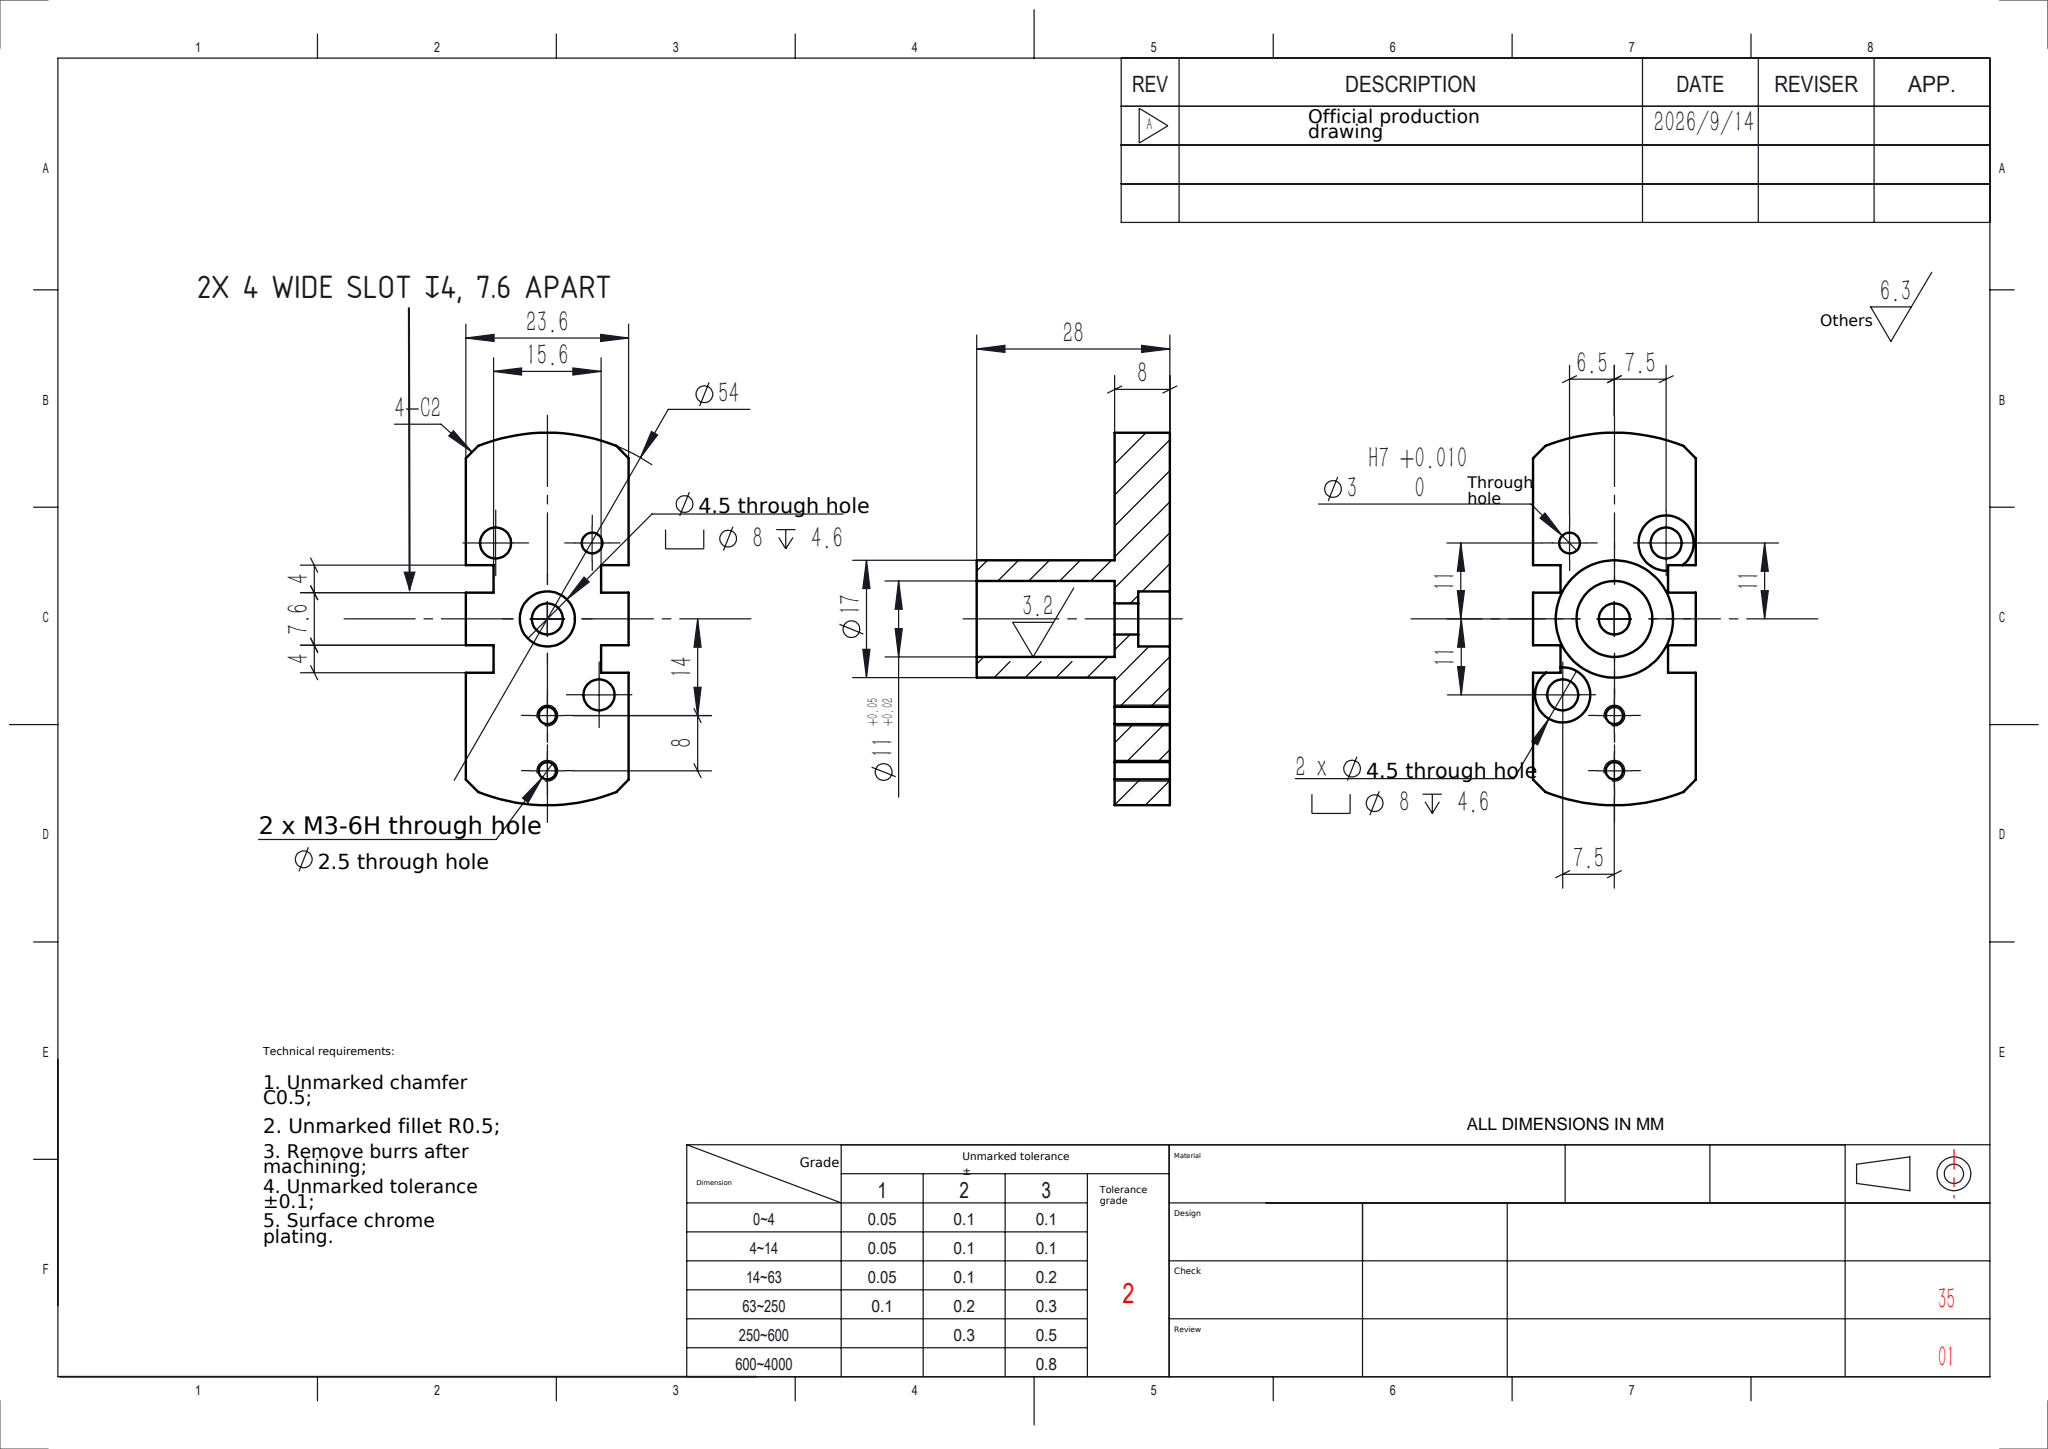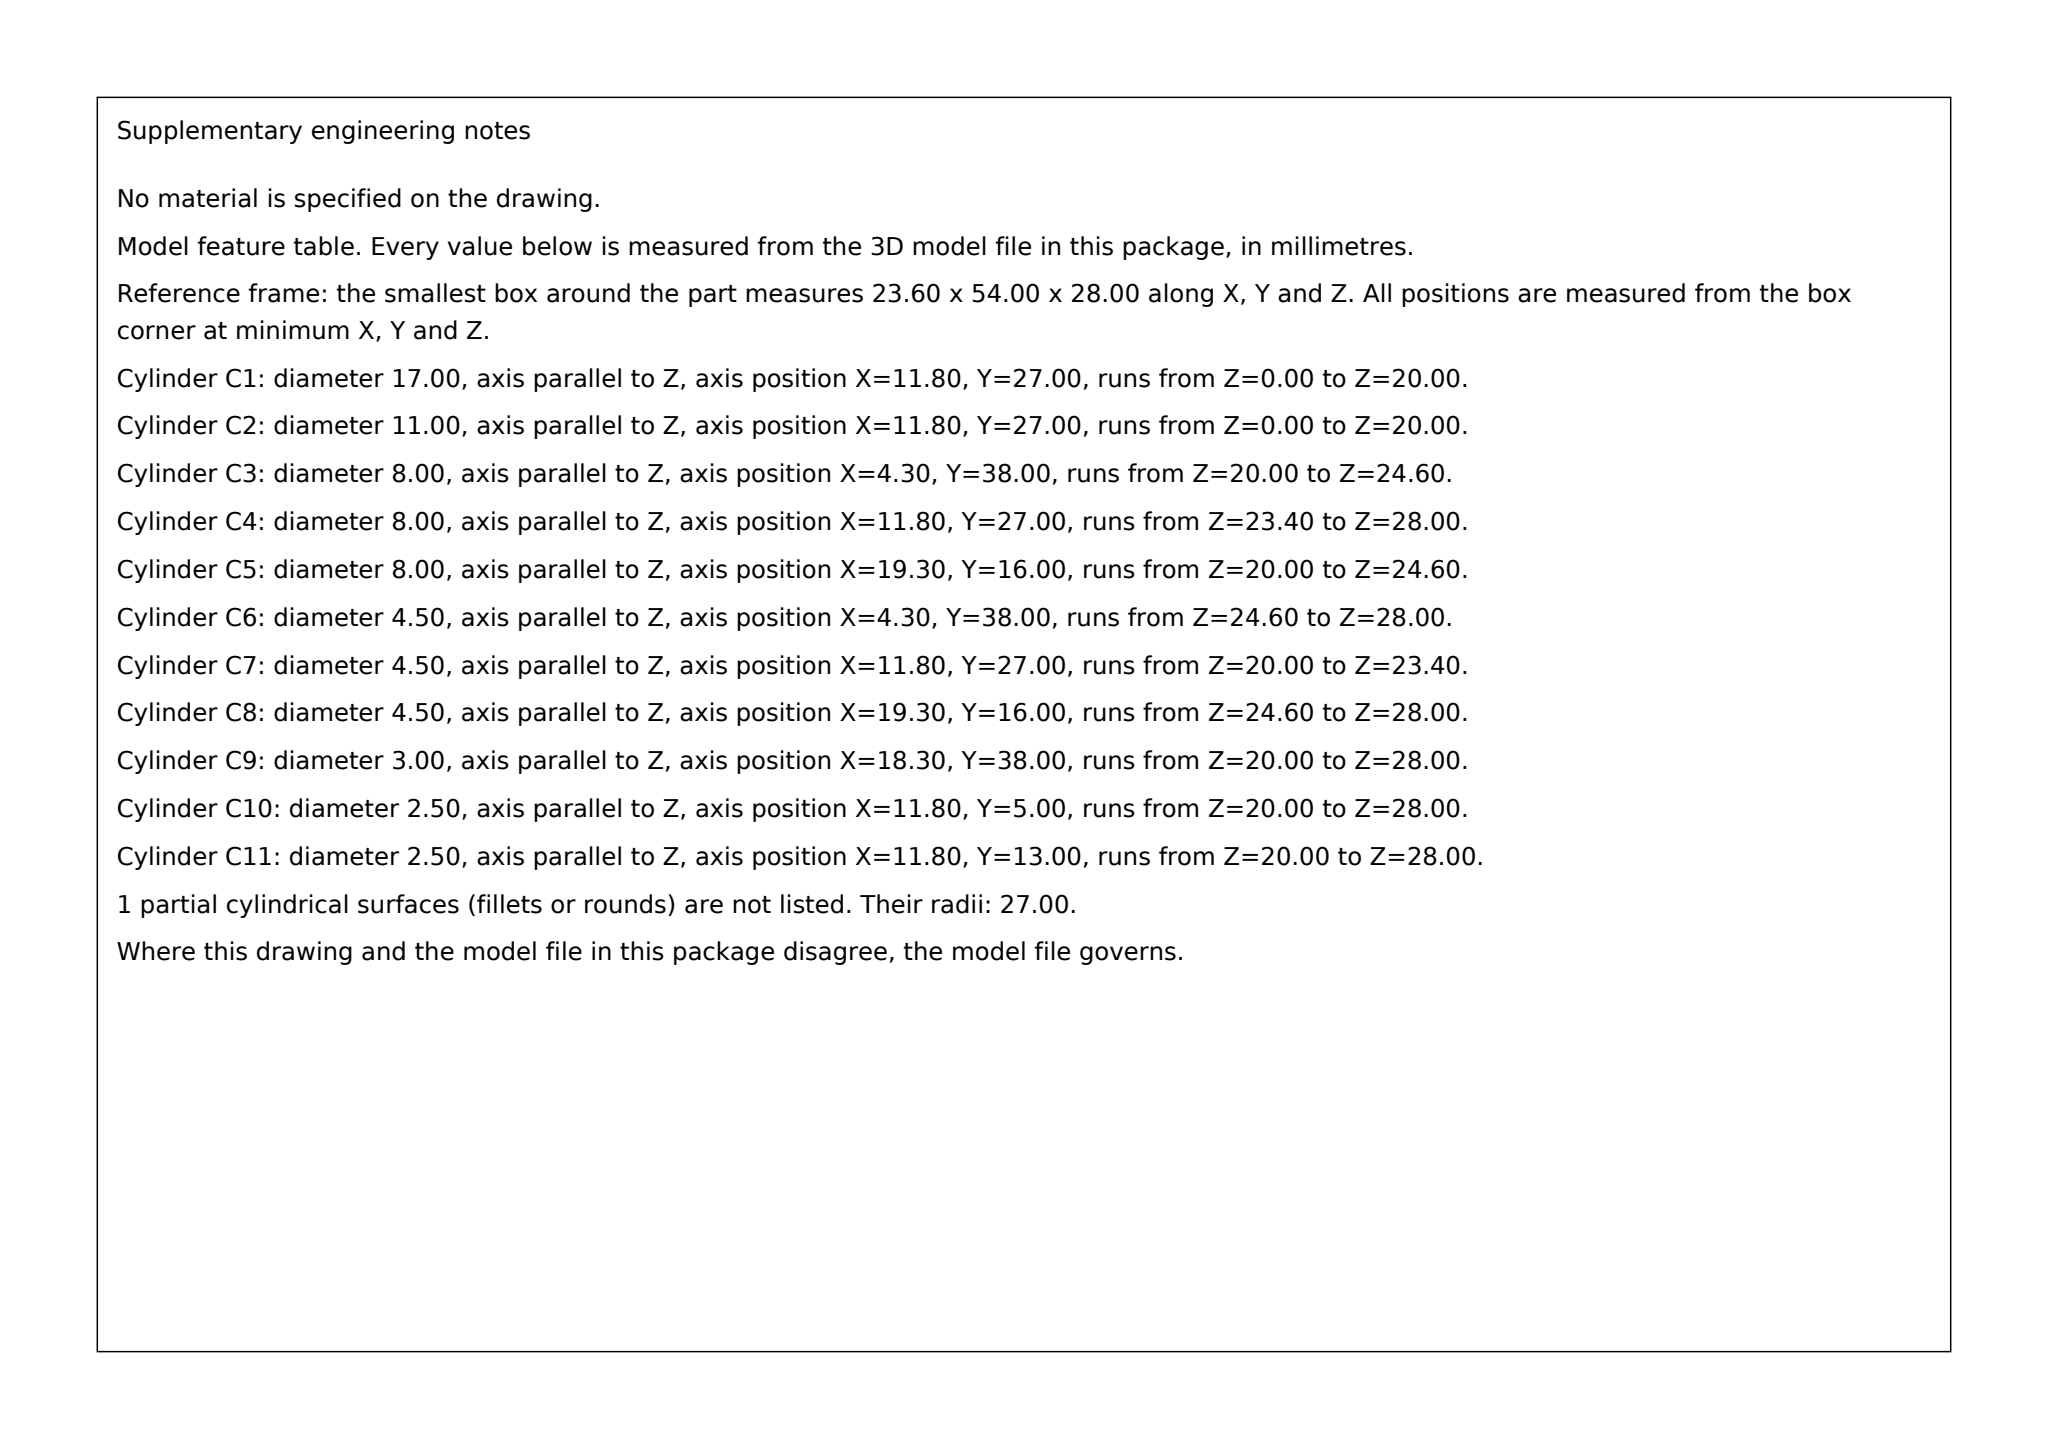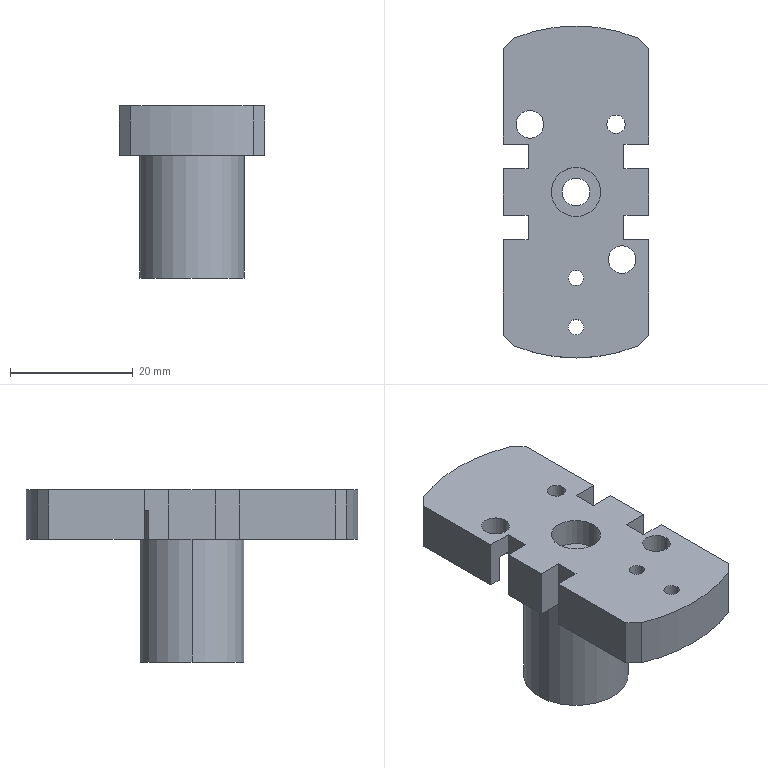Part | SolidWorks | mm | 1 solid | 55 faces | box 23.6 x 54 x 28 mm | volume 10977 mm3 | plane 29 | cylinder 26 | commonest cylinder face diameters 8 x8 4.5 x6 2.5 x4 3 x2 11 x2 17 x2 54 x2
Drawing notes:
2X SIDE SLOT 4 ±0.1 WIDE X 4 DEEP, 7.6 BETWEEN SLOTS | from the solid: Y planes 19.2/23.2 and 30.8/34.8 (4 wide, 7.6 between); X planes 0-4.0 and 19.6-23.6 (4 deep)